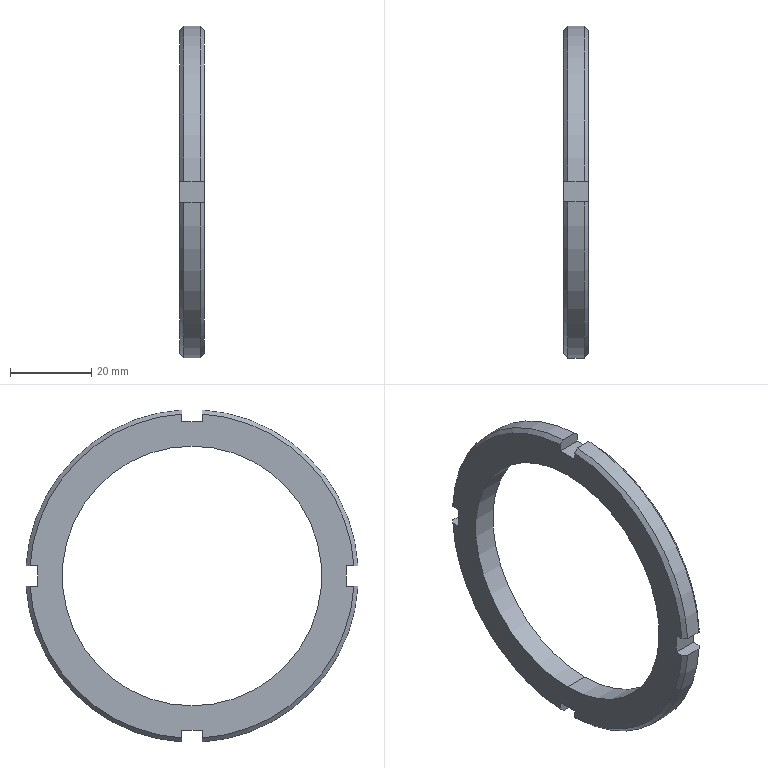Component | SolidWorks | 19LockNut-1 | 1 solid | 28 faces | box 6 x 81.85 x 81.85 mm | volume 11792 mm3 | plane 14 | cone 8 | cylinder 6 | commonest cylinder face diameters 82 x4 64 x2
build123d program:
from build123d import *

# Parameters (mm, degrees)
SKETCH9_R           = 41
BOSS_EXTRUDE3_DEPTH = 6
CHAMFER1_SIZE       = 1
SKETCH10_W          = 5
SKETCH10_H          = 19.557
CUT_EXTRUDE5_DEPTH  = 59.292
CIRPATTERN1_COUNT   = 4
M64_TAPPED_HOLE1_D  = 64


with BuildPart() as part:
    # Sketch9 → Boss-Extrude3 (new body)
    with BuildSketch(Plane(origin=(0, 0, 0), x_dir=(0, 0, -1), z_dir=(1, 0, 0))):
        Circle(SKETCH9_R)
    extrude(amount=BOSS_EXTRUDE3_DEPTH)

    # Chamfer1
    chamfer1_edges = [part.edges().sort_by_distance(p)[0] for p in [
        (0, 0, 41),
        (6, 0, 41),
    ]]
    chamfer(chamfer1_edges, length=CHAMFER1_SIZE)

    # Sketch10 → Cut-Extrude5 (cut, through all)
    with BuildSketch(Plane(origin=(6, 0, 0), x_dir=(0, 0, -1), z_dir=(1, 0, 0))):
        with Locations((0, 47.779)):
            Rectangle(SKETCH10_W, SKETCH10_H)
    cut_extrude5 = extrude(amount=-CUT_EXTRUDE5_DEPTH, mode=Mode.SUBTRACT)

    # CirPattern1: Cut-Extrude5 ×4 about axis
    cirpattern1_axis = Axis((0, 0, 0), (1, 0, 0))
    for i in range(1, CIRPATTERN1_COUNT):
        add(cut_extrude5.rotate(cirpattern1_axis, i * 360 / CIRPATTERN1_COUNT), mode=Mode.SUBTRACT)

    # M64 Tapped Hole1 (through all)
    with Locations(Plane(origin=(6, 0, 0), x_dir=(0, 0, -1), z_dir=(1, 0, 0))):
        with Locations((0, 0)):
            Hole(M64_TAPPED_HOLE1_D / 2)


solid = part.part

# Placed as in the assembly
solid = solid.moved(Location((-10.043, 1.776, 250), (0, 0, 0)))
STEP:
#1=CARTESIAN_POINT('',(-0.3954,0.06992,11.102));
#2=VERTEX_POINT('',#1);
#3=CARTESIAN_POINT('',(-0.3954,0.06992,8.583));
#4=VERTEX_POINT('',#3);
#5=CARTESIAN_POINT('',(-0.3954,0.06992,9.843));
#6=DIRECTION('',(1.,0.,0.));
#7=DIRECTION('',(0.,0.,-1.));
#8=AXIS2_PLACEMENT_3D('',#5,#6,#7);
#9=CIRCLE('',#8,1.26);
#10=EDGE_CURVE('',#2,#4,#9,.T.);
#11=ORIENTED_EDGE('',*,*,#10,.F.);
#12=CARTESIAN_POINT('',(-0.1592,0.06992,11.102));
#13=VERTEX_POINT('',#12);
#14=CARTESIAN_POINT('',(-0.1592,0.06992,11.102));
#15=DIRECTION('',(1.,0.,0.));
#16=VECTOR('',#15,39.37);
#17=LINE('',#14,#16);
#18=EDGE_CURVE('',#2,#13,#17,.T.);
#19=ORIENTED_EDGE('',*,*,#18,.T.);
#20=CARTESIAN_POINT('',(-0.1592,0.06992,8.583));
#21=VERTEX_POINT('',#20);
#22=CARTESIAN_POINT('',(-0.1592,0.06992,9.843));
#23=DIRECTION('',(1.,0.,0.));
#24=DIRECTION('',(0.,0.,-1.));
#25=AXIS2_PLACEMENT_3D('',#22,#23,#24);
#26=CIRCLE('',#25,1.26);
#27=EDGE_CURVE('',#13,#21,#26,.T.);
#28=ORIENTED_EDGE('',*,*,#27,.T.);
#29=CARTESIAN_POINT('',(-0.1592,0.06992,8.583));
#30=DIRECTION('',(1.,0.,0.));
#31=VECTOR('',#30,39.37);
#32=LINE('',#29,#31);
#33=EDGE_CURVE('',#4,#21,#32,.T.);
#34=ORIENTED_EDGE('',*,*,#33,.F.);
#35=EDGE_LOOP('',(#11,#19,#28,#34));
#36=FACE_OUTER_BOUND('',#35,.T.);
#37=CARTESIAN_POINT('',(-0.1592,0.06992,9.843));
#38=DIRECTION('',(1.,0.,0.));
#39=DIRECTION('',(0.,0.,-1.));
#40=AXIS2_PLACEMENT_3D('',#37,#38,#39);
#41=CYLINDRICAL_SURFACE('',#40,1.26);
#42=ADVANCED_FACE('',(#36),#41,.F.);
#43=CARTESIAN_POINT('',(-0.356,1.681,9.941));
#44=VERTEX_POINT('',#43);
#45=CARTESIAN_POINT('',(-0.356,0.1683,11.454));
#46=VERTEX_POINT('',#45);
#47=CARTESIAN_POINT('',(-0.356,0.06992,9.843));
#48=DIRECTION('',(1.,0.,0.));
#49=DIRECTION('',(0.,0.,-1.));
#50=AXIS2_PLACEMENT_3D('',#47,#48,#49);
#51=CIRCLE('',#50,1.614);
#52=EDGE_CURVE('',#44,#46,#51,.T.);
#53=ORIENTED_EDGE('',*,*,#52,.T.);
#54=CARTESIAN_POINT('',(-0.1985,0.1683,11.454));
#55=VERTEX_POINT('',#54);
#56=CARTESIAN_POINT('',(-0.1592,0.1683,11.454));
#57=DIRECTION('',(1.,0.,0.));
#58=VECTOR('',#57,39.37);
#59=LINE('',#56,#58);
#60=EDGE_CURVE('',#46,#55,#59,.T.);
#61=ORIENTED_EDGE('',*,*,#60,.T.);
#62=CARTESIAN_POINT('',(-0.1985,1.681,9.941));
#63=VERTEX_POINT('',#62);
#64=CARTESIAN_POINT('',(-0.1985,0.06992,9.843));
#65=DIRECTION('',(-1.,0.,0.));
#66=DIRECTION('',(0.,0.,-1.));
#67=AXIS2_PLACEMENT_3D('',#64,#65,#66);
#68=CIRCLE('',#67,1.614);
#69=EDGE_CURVE('',#55,#63,#68,.T.);
#70=ORIENTED_EDGE('',*,*,#69,.T.);
#71=CARTESIAN_POINT('',(-0.1592,1.681,9.941));
#72=DIRECTION('',(-1.,0.,0.));
#73=VECTOR('',#72,39.37);
#74=LINE('',#71,#73);
#75=EDGE_CURVE('',#63,#44,#74,.T.);
#76=ORIENTED_EDGE('',*,*,#75,.T.);
#77=EDGE_LOOP('',(#53,#61,#70,#76));
#78=FACE_OUTER_BOUND('',#77,.T.);
#79=CARTESIAN_POINT('',(-0.1592,0.06992,9.843));
#80=DIRECTION('',(-1.,0.,0.));
#81=DIRECTION('',(0.,0.,1.));
#82=AXIS2_PLACEMENT_3D('',#79,#80,#81);
#83=CYLINDRICAL_SURFACE('',#82,1.614);
#84=ADVANCED_FACE('',(#78),#83,.T.);
#85=CARTESIAN_POINT('',(-0.1985,-1.541,9.941));
#86=VERTEX_POINT('',#85);
#87=CARTESIAN_POINT('',(-0.1985,-0.0285,11.454));
#88=VERTEX_POINT('',#87);
#89=CARTESIAN_POINT('',(-0.1985,0.06992,9.843));
#90=DIRECTION('',(-1.,0.,0.));
#91=DIRECTION('',(0.,-0.,-1.));
#92=AXIS2_PLACEMENT_3D('',#89,#90,#91);
#93=CIRCLE('',#92,1.614);
#94=EDGE_CURVE('',#86,#88,#93,.T.);
#95=ORIENTED_EDGE('',*,*,#94,.T.);
#96=CARTESIAN_POINT('',(-0.356,-0.0285,11.454));
#97=VERTEX_POINT('',#96);
#98=CARTESIAN_POINT('',(-0.1592,-0.0285,11.454));
#99=DIRECTION('',(-1.,0.,0.));
#100=VECTOR('',#99,39.37);
#101=LINE('',#98,#100);
#102=EDGE_CURVE('',#88,#97,#101,.T.);
#103=ORIENTED_EDGE('',*,*,#102,.T.);
#104=CARTESIAN_POINT('',(-0.356,-1.541,9.941));
#105=VERTEX_POINT('',#104);
#106=CARTESIAN_POINT('',(-0.356,0.06992,9.843));
#107=DIRECTION('',(1.,0.,0.));
#108=DIRECTION('',(0.,0.,-1.));
#109=AXIS2_PLACEMENT_3D('',#106,#107,#108);
#110=CIRCLE('',#109,1.614);
#111=EDGE_CURVE('',#97,#105,#110,.T.);
#112=ORIENTED_EDGE('',*,*,#111,.T.);
#113=CARTESIAN_POINT('',(-0.1592,-1.541,9.941));
#114=DIRECTION('',(1.,0.,0.));
#115=VECTOR('',#114,39.37);
#116=LINE('',#113,#115);
#117=EDGE_CURVE('',#105,#86,#116,.T.);
#118=ORIENTED_EDGE('',*,*,#117,.T.);
#119=EDGE_LOOP('',(#95,#103,#112,#118));
#120=FACE_OUTER_BOUND('',#119,.T.);
#121=CARTESIAN_POINT('',(-0.1592,0.06992,9.843));
#122=DIRECTION('',(-1.,0.,0.));
#123=DIRECTION('',(0.,0.,1.));
#124=AXIS2_PLACEMENT_3D('',#121,#122,#123);
#125=CYLINDRICAL_SURFACE('',#124,1.614);
#126=ADVANCED_FACE('',(#120),#125,.T.);
#127=CARTESIAN_POINT('',(-0.1985,-0.0285,8.231));
#128=VERTEX_POINT('',#127);
#129=CARTESIAN_POINT('',(-0.1985,-1.541,9.744));
#130=VERTEX_POINT('',#129);
#131=CARTESIAN_POINT('',(-0.1985,0.06992,9.843));
#132=DIRECTION('',(-1.,0.,0.));
#133=DIRECTION('',(0.,0.,-1.));
#134=AXIS2_PLACEMENT_3D('',#131,#132,#133);
#135=CIRCLE('',#134,1.614);
#136=EDGE_CURVE('',#128,#130,#135,.T.);
#137=ORIENTED_EDGE('',*,*,#136,.T.);
#138=CARTESIAN_POINT('',(-0.356,-1.541,9.744));
#139=VERTEX_POINT('',#138);
#140=CARTESIAN_POINT('',(-0.1592,-1.541,9.744));
#141=DIRECTION('',(-1.,0.,0.));
#142=VECTOR('',#141,39.37);
#143=LINE('',#140,#142);
#144=EDGE_CURVE('',#130,#139,#143,.T.);
#145=ORIENTED_EDGE('',*,*,#144,.T.);
#146=CARTESIAN_POINT('',(-0.356,-0.0285,8.231));
#147=VERTEX_POINT('',#146);
#148=CARTESIAN_POINT('',(-0.356,0.06992,9.843));
#149=DIRECTION('',(1.,0.,0.));
#150=DIRECTION('',(0.,0.,-1.));
#151=AXIS2_PLACEMENT_3D('',#148,#149,#150);
#152=CIRCLE('',#151,1.614);
#153=EDGE_CURVE('',#139,#147,#152,.T.);
#154=ORIENTED_EDGE('',*,*,#153,.T.);
#155=CARTESIAN_POINT('',(-0.1592,-0.0285,8.231));
#156=DIRECTION('',(1.,0.,0.));
#157=VECTOR('',#156,39.37);
#158=LINE('',#155,#157);
#159=EDGE_CURVE('',#147,#128,#158,.T.);
#160=ORIENTED_EDGE('',*,*,#159,.T.);
#161=EDGE_LOOP('',(#137,#145,#154,#160));
#162=FACE_OUTER_BOUND('',#161,.T.);
#163=CARTESIAN_POINT('',(-0.1592,0.06992,9.843));
#164=DIRECTION('',(-1.,0.,0.));
#165=DIRECTION('',(0.,0.,1.));
#166=AXIS2_PLACEMENT_3D('',#163,#164,#165);
#167=CYLINDRICAL_SURFACE('',#166,1.614);
#168=ADVANCED_FACE('',(#162),#167,.T.);
#169=CARTESIAN_POINT('',(-0.3954,0.1683,11.414));
#170=VERTEX_POINT('',#169);
#171=CARTESIAN_POINT('',(-0.356,0.1683,11.454));
#172=CARTESIAN_POINT('',(-0.3662,0.1683,11.444));
#173=CARTESIAN_POINT('',(-0.3763,0.1683,11.433));
#174=CARTESIAN_POINT('',(-0.3865,0.1683,11.423));
#175=CARTESIAN_POINT('',(-0.3894,0.1683,11.42));
#176=CARTESIAN_POINT('',(-0.3924,0.1683,11.417));
#177=CARTESIAN_POINT('',(-0.3954,0.1683,11.414));
#178=B_SPLINE_CURVE_WITH_KNOTS('',3,(#171,#172,#173,#174,#175,#176,#177),.UNSPECIFIED.,.F.,.F.,(4,3,4),(0.005082,0.006177,0.006497),.UNSPECIFIED.);
#179=EDGE_CURVE('',#46,#170,#178,.T.);
#180=ORIENTED_EDGE('',*,*,#179,.F.);
#181=ORIENTED_EDGE('',*,*,#52,.F.);
#182=CARTESIAN_POINT('',(-0.3954,1.642,9.941));
#183=VERTEX_POINT('',#182);
#184=CARTESIAN_POINT('',(-0.3954,1.642,9.941));
#185=CARTESIAN_POINT('',(-0.3924,1.645,9.941));
#186=CARTESIAN_POINT('',(-0.3894,1.648,9.941));
#187=CARTESIAN_POINT('',(-0.3865,1.651,9.941));
#188=CARTESIAN_POINT('',(-0.3763,1.661,9.941));
#189=CARTESIAN_POINT('',(-0.3662,1.671,9.941));
#190=CARTESIAN_POINT('',(-0.356,1.681,9.941));
#191=B_SPLINE_CURVE_WITH_KNOTS('',3,(#184,#185,#186,#187,#188,#189,#190),.UNSPECIFIED.,.F.,.F.,(4,3,4),(0.005857,0.006177,0.007273),.UNSPECIFIED.);
#192=EDGE_CURVE('',#183,#44,#191,.T.);
#193=ORIENTED_EDGE('',*,*,#192,.F.);
#194=CARTESIAN_POINT('',(-0.3954,0.06992,9.843));
#195=DIRECTION('',(-1.,0.,0.));
#196=DIRECTION('',(0.,-0.,-1.));
#197=AXIS2_PLACEMENT_3D('',#194,#195,#196);
#198=CIRCLE('',#197,1.575);
#199=EDGE_CURVE('',#170,#183,#198,.T.);
#200=ORIENTED_EDGE('',*,*,#199,.F.);
#201=EDGE_LOOP('',(#180,#181,#193,#200));
#202=FACE_OUTER_BOUND('',#201,.T.);
#203=CARTESIAN_POINT('',(-0.356,0.06992,9.843));
#204=DIRECTION('',(1.,0.,0.));
#205=DIRECTION('',(0.,0.,-1.));
#206=AXIS2_PLACEMENT_3D('',#203,#204,#205);
#207=CONICAL_SURFACE('',#206,1.614,0.7854);
#208=ADVANCED_FACE('',(#202),#207,.T.);
#209=CARTESIAN_POINT('',(-0.3954,-0.0285,11.414));
#210=VERTEX_POINT('',#209);
#211=CARTESIAN_POINT('',(-0.3954,-0.0285,11.414));
#212=CARTESIAN_POINT('',(-0.3924,-0.0285,11.417));
#213=CARTESIAN_POINT('',(-0.3894,-0.0285,11.42));
#214=CARTESIAN_POINT('',(-0.3865,-0.0285,11.423));
#215=CARTESIAN_POINT('',(-0.3763,-0.0285,11.433));
#216=CARTESIAN_POINT('',(-0.3662,-0.0285,11.444));
#217=CARTESIAN_POINT('',(-0.356,-0.0285,11.454));
#218=B_SPLINE_CURVE_WITH_KNOTS('',3,(#211,#212,#213,#214,#215,#216,#217),.UNSPECIFIED.,.F.,.F.,(4,3,4),(0.005857,0.006177,0.007273),.UNSPECIFIED.);
#219=EDGE_CURVE('',#210,#97,#218,.T.);
#220=ORIENTED_EDGE('',*,*,#219,.F.);
#221=CARTESIAN_POINT('',(-0.3954,-1.502,9.941));
#222=VERTEX_POINT('',#221);
#223=CARTESIAN_POINT('',(-0.3954,0.06992,9.843));
#224=DIRECTION('',(-1.,0.,0.));
#225=DIRECTION('',(0.,0.,-1.));
#226=AXIS2_PLACEMENT_3D('',#223,#224,#225);
#227=CIRCLE('',#226,1.575);
#228=EDGE_CURVE('',#222,#210,#227,.T.);
#229=ORIENTED_EDGE('',*,*,#228,.F.);
#230=CARTESIAN_POINT('',(-0.356,-1.541,9.941));
#231=CARTESIAN_POINT('',(-0.3612,-1.536,9.941));
#232=CARTESIAN_POINT('',(-0.3665,-1.531,9.941));
#233=CARTESIAN_POINT('',(-0.3717,-1.526,9.941));
#234=CARTESIAN_POINT('',(-0.3796,-1.518,9.941));
#235=CARTESIAN_POINT('',(-0.3875,-1.51,9.941));
#236=CARTESIAN_POINT('',(-0.3954,-1.502,9.941));
#237=B_SPLINE_CURVE_WITH_KNOTS('',3,(#230,#231,#232,#233,#234,#235,#236),.UNSPECIFIED.,.F.,.F.,(4,3,4),(0.005613,0.006177,0.007028),.UNSPECIFIED.);
#238=EDGE_CURVE('',#105,#222,#237,.T.);
#239=ORIENTED_EDGE('',*,*,#238,.F.);
#240=ORIENTED_EDGE('',*,*,#111,.F.);
#241=EDGE_LOOP('',(#220,#229,#239,#240));
#242=FACE_OUTER_BOUND('',#241,.T.);
#243=CARTESIAN_POINT('',(-0.356,0.06992,9.843));
#244=DIRECTION('',(1.,0.,0.));
#245=DIRECTION('',(0.,0.,-1.));
#246=AXIS2_PLACEMENT_3D('',#243,#244,#245);
#247=CONICAL_SURFACE('',#246,1.614,0.7854);
#248=ADVANCED_FACE('',(#242),#247,.T.);
#249=CARTESIAN_POINT('',(-0.3954,-1.502,9.744));
#250=VERTEX_POINT('',#249);
#251=CARTESIAN_POINT('',(-0.3954,-1.502,9.744));
#252=CARTESIAN_POINT('',(-0.3875,-1.51,9.744));
#253=CARTESIAN_POINT('',(-0.3796,-1.518,9.744));
#254=CARTESIAN_POINT('',(-0.3717,-1.526,9.744));
#255=CARTESIAN_POINT('',(-0.3665,-1.531,9.744));
#256=CARTESIAN_POINT('',(-0.3612,-1.536,9.744));
#257=CARTESIAN_POINT('',(-0.356,-1.541,9.744));
#258=B_SPLINE_CURVE_WITH_KNOTS('',3,(#251,#252,#253,#254,#255,#256,#257),.UNSPECIFIED.,.F.,.F.,(4,3,4),(0.005326,0.006177,0.006742),.UNSPECIFIED.);
#259=EDGE_CURVE('',#250,#139,#258,.T.);
#260=ORIENTED_EDGE('',*,*,#259,.F.);
#261=CARTESIAN_POINT('',(-0.3954,-0.0285,8.271));
#262=VERTEX_POINT('',#261);
#263=CARTESIAN_POINT('',(-0.3954,0.06992,9.843));
#264=DIRECTION('',(-1.,0.,0.));
#265=DIRECTION('',(0.,0.,-1.));
#266=AXIS2_PLACEMENT_3D('',#263,#264,#265);
#267=CIRCLE('',#266,1.575);
#268=EDGE_CURVE('',#262,#250,#267,.T.);
#269=ORIENTED_EDGE('',*,*,#268,.F.);
#270=CARTESIAN_POINT('',(-0.356,-0.0285,8.231));
#271=CARTESIAN_POINT('',(-0.3612,-0.0285,8.237));
#272=CARTESIAN_POINT('',(-0.3665,-0.0285,8.242));
#273=CARTESIAN_POINT('',(-0.3717,-0.0285,8.247));
#274=CARTESIAN_POINT('',(-0.3796,-0.0285,8.255));
#275=CARTESIAN_POINT('',(-0.3875,-0.0285,8.263));
#276=CARTESIAN_POINT('',(-0.3954,-0.0285,8.271));
#277=B_SPLINE_CURVE_WITH_KNOTS('',3,(#270,#271,#272,#273,#274,#275,#276),.UNSPECIFIED.,.F.,.F.,(4,3,4),(0.005613,0.006177,0.007028),.UNSPECIFIED.);
#278=EDGE_CURVE('',#147,#262,#277,.T.);
#279=ORIENTED_EDGE('',*,*,#278,.F.);
#280=ORIENTED_EDGE('',*,*,#153,.F.);
#281=EDGE_LOOP('',(#260,#269,#279,#280));
#282=FACE_OUTER_BOUND('',#281,.T.);
#283=CARTESIAN_POINT('',(-0.356,0.06992,9.843));
#284=DIRECTION('',(1.,0.,0.));
#285=DIRECTION('',(0.,0.,-1.));
#286=AXIS2_PLACEMENT_3D('',#283,#284,#285);
#287=CONICAL_SURFACE('',#286,1.614,0.7854);
#288=ADVANCED_FACE('',(#282),#287,.T.);
#289=CARTESIAN_POINT('',(-0.1592,0.1683,11.414));
#290=VERTEX_POINT('',#289);
#291=CARTESIAN_POINT('',(-0.1592,0.1683,11.414));
#292=CARTESIAN_POINT('',(-0.1621,0.1683,11.417));
#293=CARTESIAN_POINT('',(-0.1651,0.1683,11.42));
#294=CARTESIAN_POINT('',(-0.1681,0.1683,11.423));
#295=CARTESIAN_POINT('',(-0.1782,0.1683,11.433));
#296=CARTESIAN_POINT('',(-0.1884,0.1683,11.444));
#297=CARTESIAN_POINT('',(-0.1985,0.1683,11.454));
#298=B_SPLINE_CURVE_WITH_KNOTS('',3,(#291,#292,#293,#294,#295,#296,#297),.UNSPECIFIED.,.F.,.F.,(4,3,4),(0.005857,0.006177,0.007273),.UNSPECIFIED.);
#299=EDGE_CURVE('',#290,#55,#298,.T.);
#300=ORIENTED_EDGE('',*,*,#299,.F.);
#301=CARTESIAN_POINT('',(-0.1592,1.642,9.941));
#302=VERTEX_POINT('',#301);
#303=CARTESIAN_POINT('',(-0.1592,0.06992,9.843));
#304=DIRECTION('',(1.,0.,0.));
#305=DIRECTION('',(0.,0.,-1.));
#306=AXIS2_PLACEMENT_3D('',#303,#304,#305);
#307=CIRCLE('',#306,1.575);
#308=EDGE_CURVE('',#302,#290,#307,.T.);
#309=ORIENTED_EDGE('',*,*,#308,.F.);
#310=CARTESIAN_POINT('',(-0.1985,1.681,9.941));
#311=CARTESIAN_POINT('',(-0.1884,1.671,9.941));
#312=CARTESIAN_POINT('',(-0.1782,1.661,9.941));
#313=CARTESIAN_POINT('',(-0.1681,1.651,9.941));
#314=CARTESIAN_POINT('',(-0.1651,1.648,9.941));
#315=CARTESIAN_POINT('',(-0.1621,1.645,9.941));
#316=CARTESIAN_POINT('',(-0.1592,1.642,9.941));
#317=B_SPLINE_CURVE_WITH_KNOTS('',3,(#310,#311,#312,#313,#314,#315,#316),.UNSPECIFIED.,.F.,.F.,(4,3,4),(0.005082,0.006177,0.006497),.UNSPECIFIED.);
#318=EDGE_CURVE('',#63,#302,#317,.T.);
#319=ORIENTED_EDGE('',*,*,#318,.F.);
#320=ORIENTED_EDGE('',*,*,#69,.F.);
#321=EDGE_LOOP('',(#300,#309,#319,#320));
#322=FACE_OUTER_BOUND('',#321,.T.);
#323=CARTESIAN_POINT('',(-0.1592,0.06992,9.843));
#324=DIRECTION('',(-1.,0.,0.));
#325=DIRECTION('',(0.,0.,1.));
#326=AXIS2_PLACEMENT_3D('',#323,#324,#325);
#327=CONICAL_SURFACE('',#326,1.575,0.7854);
#328=ADVANCED_FACE('',(#322),#327,.T.);
#329=CARTESIAN_POINT('',(-0.1592,-0.0285,11.414));
#330=VERTEX_POINT('',#329);
#331=CARTESIAN_POINT('',(-0.1985,-0.0285,11.454));
#332=CARTESIAN_POINT('',(-0.1884,-0.0285,11.444));
#333=CARTESIAN_POINT('',(-0.1782,-0.0285,11.433));
#334=CARTESIAN_POINT('',(-0.1681,-0.0285,11.423));
#335=CARTESIAN_POINT('',(-0.1651,-0.0285,11.42));
#336=CARTESIAN_POINT('',(-0.1621,-0.0285,11.417));
#337=CARTESIAN_POINT('',(-0.1592,-0.0285,11.414));
#338=B_SPLINE_CURVE_WITH_KNOTS('',3,(#331,#332,#333,#334,#335,#336,#337),.UNSPECIFIED.,.F.,.F.,(4,3,4),(0.005082,0.006177,0.006497),.UNSPECIFIED.);
#339=EDGE_CURVE('',#88,#330,#338,.T.);
#340=ORIENTED_EDGE('',*,*,#339,.F.);
#341=ORIENTED_EDGE('',*,*,#94,.F.);
#342=CARTESIAN_POINT('',(-0.1592,-1.502,9.941));
#343=VERTEX_POINT('',#342);
#344=CARTESIAN_POINT('',(-0.1592,-1.502,9.941));
#345=CARTESIAN_POINT('',(-0.1671,-1.51,9.941));
#346=CARTESIAN_POINT('',(-0.1749,-1.518,9.941));
#347=CARTESIAN_POINT('',(-0.1828,-1.526,9.941));
#348=CARTESIAN_POINT('',(-0.1881,-1.531,9.941));
#349=CARTESIAN_POINT('',(-0.1933,-1.536,9.941));
#350=CARTESIAN_POINT('',(-0.1985,-1.541,9.941));
#351=B_SPLINE_CURVE_WITH_KNOTS('',3,(#344,#345,#346,#347,#348,#349,#350),.UNSPECIFIED.,.F.,.F.,(4,3,4),(0.005326,0.006177,0.006742),.UNSPECIFIED.);
#352=EDGE_CURVE('',#343,#86,#351,.T.);
#353=ORIENTED_EDGE('',*,*,#352,.F.);
#354=CARTESIAN_POINT('',(-0.1592,0.06992,9.843));
#355=DIRECTION('',(1.,0.,0.));
#356=DIRECTION('',(0.,0.,-1.));
#357=AXIS2_PLACEMENT_3D('',#354,#355,#356);
#358=CIRCLE('',#357,1.575);
#359=EDGE_CURVE('',#330,#343,#358,.T.);
#360=ORIENTED_EDGE('',*,*,#359,.F.);
#361=EDGE_LOOP('',(#340,#341,#353,#360));
#362=FACE_OUTER_BOUND('',#361,.T.);
#363=CARTESIAN_POINT('',(-0.1592,0.06992,9.843));
#364=DIRECTION('',(-1.,0.,0.));
#365=DIRECTION('',(0.,0.,1.));
#366=AXIS2_PLACEMENT_3D('',#363,#364,#365);
#367=CONICAL_SURFACE('',#366,1.575,0.7854);
#368=ADVANCED_FACE('',(#362),#367,.T.);
#369=CARTESIAN_POINT('',(-0.1592,-1.502,9.744));
#370=VERTEX_POINT('',#369);
#371=CARTESIAN_POINT('',(-0.1985,-1.541,9.744));
#372=CARTESIAN_POINT('',(-0.1933,-1.536,9.744));
#373=CARTESIAN_POINT('',(-0.1881,-1.531,9.744));
#374=CARTESIAN_POINT('',(-0.1828,-1.526,9.744));
#375=CARTESIAN_POINT('',(-0.1749,-1.518,9.744));
#376=CARTESIAN_POINT('',(-0.1671,-1.51,9.744));
#377=CARTESIAN_POINT('',(-0.1592,-1.502,9.744));
#378=B_SPLINE_CURVE_WITH_KNOTS('',3,(#371,#372,#373,#374,#375,#376,#377),.UNSPECIFIED.,.F.,.F.,(4,3,4),(0.005613,0.006177,0.007028),.UNSPECIFIED.);
#379=EDGE_CURVE('',#130,#370,#378,.T.);
#380=ORIENTED_EDGE('',*,*,#379,.F.);
#381=ORIENTED_EDGE('',*,*,#136,.F.);
#382=CARTESIAN_POINT('',(-0.1592,-0.0285,8.271));
#383=VERTEX_POINT('',#382);
#384=CARTESIAN_POINT('',(-0.1592,-0.0285,8.271));
#385=CARTESIAN_POINT('',(-0.1671,-0.0285,8.263));
#386=CARTESIAN_POINT('',(-0.1749,-0.0285,8.255));
#387=CARTESIAN_POINT('',(-0.1828,-0.0285,8.247));
#388=CARTESIAN_POINT('',(-0.1881,-0.0285,8.242));
#389=CARTESIAN_POINT('',(-0.1933,-0.0285,8.237));
#390=CARTESIAN_POINT('',(-0.1985,-0.0285,8.231));
#391=B_SPLINE_CURVE_WITH_KNOTS('',3,(#384,#385,#386,#387,#388,#389,#390),.UNSPECIFIED.,.F.,.F.,(4,3,4),(0.005326,0.006177,0.006742),.UNSPECIFIED.);
#392=EDGE_CURVE('',#383,#128,#391,.T.);
#393=ORIENTED_EDGE('',*,*,#392,.F.);
#394=CARTESIAN_POINT('',(-0.1592,0.06992,9.843));
#395=DIRECTION('',(1.,0.,0.));
#396=DIRECTION('',(0.,0.,-1.));
#397=AXIS2_PLACEMENT_3D('',#394,#395,#396);
#398=CIRCLE('',#397,1.575);
#399=EDGE_CURVE('',#370,#383,#398,.T.);
#400=ORIENTED_EDGE('',*,*,#399,.F.);
#401=EDGE_LOOP('',(#380,#381,#393,#400));
#402=FACE_OUTER_BOUND('',#401,.T.);
#403=CARTESIAN_POINT('',(-0.1592,0.06992,9.843));
#404=DIRECTION('',(-1.,0.,0.));
#405=DIRECTION('',(0.,0.,1.));
#406=AXIS2_PLACEMENT_3D('',#403,#404,#405);
#407=CONICAL_SURFACE('',#406,1.575,0.7854);
#408=ADVANCED_FACE('',(#402),#407,.T.);
#409=CARTESIAN_POINT('',(-0.1985,1.681,9.744));
#410=VERTEX_POINT('',#409);
#411=CARTESIAN_POINT('',(-0.1985,0.1683,8.231));
#412=VERTEX_POINT('',#411);
#413=CARTESIAN_POINT('',(-0.1985,0.06992,9.843));
#414=DIRECTION('',(-1.,0.,0.));
#415=DIRECTION('',(0.,-0.,-1.));
#416=AXIS2_PLACEMENT_3D('',#413,#414,#415);
#417=CIRCLE('',#416,1.614);
#418=EDGE_CURVE('',#410,#412,#417,.T.);
#419=ORIENTED_EDGE('',*,*,#418,.T.);
#420=CARTESIAN_POINT('',(-0.356,0.1683,8.231));
#421=VERTEX_POINT('',#420);
#422=CARTESIAN_POINT('',(-0.1592,0.1683,8.231));
#423=DIRECTION('',(-1.,0.,0.));
#424=VECTOR('',#423,39.37);
#425=LINE('',#422,#424);
#426=EDGE_CURVE('',#412,#421,#425,.T.);
#427=ORIENTED_EDGE('',*,*,#426,.T.);
#428=CARTESIAN_POINT('',(-0.356,1.681,9.744));
#429=VERTEX_POINT('',#428);
#430=CARTESIAN_POINT('',(-0.356,0.06992,9.843));
#431=DIRECTION('',(1.,0.,0.));
#432=DIRECTION('',(0.,0.,-1.));
#433=AXIS2_PLACEMENT_3D('',#430,#431,#432);
#434=CIRCLE('',#433,1.614);
#435=EDGE_CURVE('',#421,#429,#434,.T.);
#436=ORIENTED_EDGE('',*,*,#435,.T.);
#437=CARTESIAN_POINT('',(-0.1592,1.681,9.744));
#438=DIRECTION('',(1.,0.,0.));
#439=VECTOR('',#438,39.37);
#440=LINE('',#437,#439);
#441=EDGE_CURVE('',#429,#410,#440,.T.);
#442=ORIENTED_EDGE('',*,*,#441,.T.);
#443=EDGE_LOOP('',(#419,#427,#436,#442));
#444=FACE_OUTER_BOUND('',#443,.T.);
#445=CARTESIAN_POINT('',(-0.1592,0.06992,9.843));
#446=DIRECTION('',(-1.,0.,0.));
#447=DIRECTION('',(0.,0.,1.));
#448=AXIS2_PLACEMENT_3D('',#445,#446,#447);
#449=CYLINDRICAL_SURFACE('',#448,1.614);
#450=ADVANCED_FACE('',(#444),#449,.T.);
#451=CARTESIAN_POINT('',(-0.1592,0.06992,9.843));
#452=DIRECTION('',(1.,0.,0.));
#453=DIRECTION('',(0.,0.,-1.));
#454=AXIS2_PLACEMENT_3D('',#451,#452,#453);
#455=CIRCLE('',#454,1.26);
#456=EDGE_CURVE('',#21,#13,#455,.T.);
#457=ORIENTED_EDGE('',*,*,#456,.F.);
#458=ORIENTED_EDGE('',*,*,#27,.F.);
#459=EDGE_LOOP('',(#457,#458));
#460=FACE_BOUND('',#459,.T.);
#461=CARTESIAN_POINT('',(-0.1592,0.1683,11.339));
#462=VERTEX_POINT('',#461);
#463=CARTESIAN_POINT('',(-0.1592,0.1683,12.109));
#464=DIRECTION('',(0.,-0.,1.));
#465=VECTOR('',#464,39.37);
#466=LINE('',#463,#465);
#467=EDGE_CURVE('',#462,#290,#466,.T.);
#468=ORIENTED_EDGE('',*,*,#467,.F.);
#469=CARTESIAN_POINT('',(-0.1592,-0.0285,11.339));
#470=VERTEX_POINT('',#469);
#471=CARTESIAN_POINT('',(-0.1592,-0.0285,11.339));
#472=DIRECTION('',(0.,1.,0.));
#473=VECTOR('',#472,39.37);
#474=LINE('',#471,#473);
#475=EDGE_CURVE('',#470,#462,#474,.T.);
#476=ORIENTED_EDGE('',*,*,#475,.F.);
#477=CARTESIAN_POINT('',(-0.1592,-0.0285,12.109));
#478=DIRECTION('',(0.,0.,-1.));
#479=VECTOR('',#478,39.37);
#480=LINE('',#477,#479);
#481=EDGE_CURVE('',#330,#470,#480,.T.);
#482=ORIENTED_EDGE('',*,*,#481,.F.);
#483=ORIENTED_EDGE('',*,*,#359,.T.);
#484=CARTESIAN_POINT('',(-0.1592,-1.426,9.941));
#485=VERTEX_POINT('',#484);
#486=CARTESIAN_POINT('',(-0.1592,-2.196,9.941));
#487=DIRECTION('',(0.,-1.,0.));
#488=VECTOR('',#487,39.37);
#489=LINE('',#486,#488);
#490=EDGE_CURVE('',#485,#343,#489,.T.);
#491=ORIENTED_EDGE('',*,*,#490,.F.);
#492=CARTESIAN_POINT('',(-0.1592,-1.426,9.744));
#493=VERTEX_POINT('',#492);
#494=CARTESIAN_POINT('',(-0.1592,-1.426,9.744));
#495=DIRECTION('',(0.,0.,1.));
#496=VECTOR('',#495,39.37);
#497=LINE('',#494,#496);
#498=EDGE_CURVE('',#493,#485,#497,.T.);
#499=ORIENTED_EDGE('',*,*,#498,.F.);
#500=CARTESIAN_POINT('',(-0.1592,-2.196,9.744));
#501=DIRECTION('',(0.,1.,0.));
#502=VECTOR('',#501,39.37);
#503=LINE('',#500,#502);
#504=EDGE_CURVE('',#370,#493,#503,.T.);
#505=ORIENTED_EDGE('',*,*,#504,.F.);
#506=ORIENTED_EDGE('',*,*,#399,.T.);
#507=CARTESIAN_POINT('',(-0.1592,-0.0285,8.346));
#508=VERTEX_POINT('',#507);
#509=CARTESIAN_POINT('',(-0.1592,-0.0285,7.576));
#510=DIRECTION('',(0.,0.,-1.));
#511=VECTOR('',#510,39.37);
#512=LINE('',#509,#511);
#513=EDGE_CURVE('',#508,#383,#512,.T.);
#514=ORIENTED_EDGE('',*,*,#513,.F.);
#515=CARTESIAN_POINT('',(-0.1592,0.1683,8.346));
#516=VERTEX_POINT('',#515);
#517=CARTESIAN_POINT('',(-0.1592,0.1683,8.346));
#518=DIRECTION('',(0.,-1.,-0.));
#519=VECTOR('',#518,39.37);
#520=LINE('',#517,#519);
#521=EDGE_CURVE('',#516,#508,#520,.T.);
#522=ORIENTED_EDGE('',*,*,#521,.F.);
#523=CARTESIAN_POINT('',(-0.1592,0.1683,8.271));
#524=VERTEX_POINT('',#523);
#525=CARTESIAN_POINT('',(-0.1592,0.1683,7.576));
#526=DIRECTION('',(0.,-0.,1.));
#527=VECTOR('',#526,39.37);
#528=LINE('',#525,#527);
#529=EDGE_CURVE('',#524,#516,#528,.T.);
#530=ORIENTED_EDGE('',*,*,#529,.F.);
#531=CARTESIAN_POINT('',(-0.1592,1.642,9.744));
#532=VERTEX_POINT('',#531);
#533=CARTESIAN_POINT('',(-0.1592,0.06992,9.843));
#534=DIRECTION('',(1.,0.,0.));
#535=DIRECTION('',(0.,0.,-1.));
#536=AXIS2_PLACEMENT_3D('',#533,#534,#535);
#537=CIRCLE('',#536,1.575);
#538=EDGE_CURVE('',#524,#532,#537,.T.);
#539=ORIENTED_EDGE('',*,*,#538,.T.);
#540=CARTESIAN_POINT('',(-0.1592,1.566,9.744));
#541=VERTEX_POINT('',#540);
#542=CARTESIAN_POINT('',(-0.1592,2.336,9.744));
#543=DIRECTION('',(0.,1.,0.));
#544=VECTOR('',#543,39.37);
#545=LINE('',#542,#544);
#546=EDGE_CURVE('',#541,#532,#545,.T.);
#547=ORIENTED_EDGE('',*,*,#546,.F.);
#548=CARTESIAN_POINT('',(-0.1592,1.566,9.941));
#549=VERTEX_POINT('',#548);
#550=CARTESIAN_POINT('',(-0.1592,1.566,9.941));
#551=DIRECTION('',(0.,0.,-1.));
#552=VECTOR('',#551,39.37);
#553=LINE('',#550,#552);
#554=EDGE_CURVE('',#549,#541,#553,.T.);
#555=ORIENTED_EDGE('',*,*,#554,.F.);
#556=CARTESIAN_POINT('',(-0.1592,2.336,9.941));
#557=DIRECTION('',(0.,-1.,0.));
#558=VECTOR('',#557,39.37);
#559=LINE('',#556,#558);
#560=EDGE_CURVE('',#302,#549,#559,.T.);
#561=ORIENTED_EDGE('',*,*,#560,.F.);
#562=ORIENTED_EDGE('',*,*,#308,.T.);
#563=EDGE_LOOP('',(#468,#476,#482,#483,#491,#499,#505,#506,#514,#522,#530,#539,#547,#555,#561,#562));
#564=FACE_OUTER_BOUND('',#563,.T.);
#565=CARTESIAN_POINT('',(-0.1592,0.06992,9.843));
#566=DIRECTION('',(1.,0.,0.));
#567=DIRECTION('',(0.,0.,-1.));
#568=AXIS2_PLACEMENT_3D('',#565,#566,#567);
#569=PLANE('',#568);
#570=ADVANCED_FACE('',(#460,#564),#569,.T.);
#571=CARTESIAN_POINT('',(-0.3954,0.06992,9.843));
#572=DIRECTION('',(1.,0.,0.));
#573=DIRECTION('',(0.,0.,-1.));
#574=AXIS2_PLACEMENT_3D('',#571,#572,#573);
#575=CIRCLE('',#574,1.26);
#576=EDGE_CURVE('',#4,#2,#575,.T.);
#577=ORIENTED_EDGE('',*,*,#576,.T.);
#578=ORIENTED_EDGE('',*,*,#10,.T.);
#579=EDGE_LOOP('',(#577,#578));
#580=FACE_BOUND('',#579,.T.);
#581=CARTESIAN_POINT('',(-0.3954,-0.0285,11.339));
#582=VERTEX_POINT('',#581);
#583=CARTESIAN_POINT('',(-0.3954,0.1683,11.339));
#584=VERTEX_POINT('',#583);
#585=CARTESIAN_POINT('',(-0.3954,-0.0285,11.339));
#586=DIRECTION('',(0.,1.,0.));
#587=VECTOR('',#586,39.37);
#588=LINE('',#585,#587);
#589=EDGE_CURVE('',#582,#584,#588,.T.);
#590=ORIENTED_EDGE('',*,*,#589,.T.);
#591=CARTESIAN_POINT('',(-0.3954,0.1683,12.109));
#592=DIRECTION('',(0.,-0.,1.));
#593=VECTOR('',#592,39.37);
#594=LINE('',#591,#593);
#595=EDGE_CURVE('',#584,#170,#594,.T.);
#596=ORIENTED_EDGE('',*,*,#595,.T.);
#597=ORIENTED_EDGE('',*,*,#199,.T.);
#598=CARTESIAN_POINT('',(-0.3954,1.566,9.941));
#599=VERTEX_POINT('',#598);
#600=CARTESIAN_POINT('',(-0.3954,2.336,9.941));
#601=DIRECTION('',(0.,-1.,0.));
#602=VECTOR('',#601,39.37);
#603=LINE('',#600,#602);
#604=EDGE_CURVE('',#183,#599,#603,.T.);
#605=ORIENTED_EDGE('',*,*,#604,.T.);
#606=CARTESIAN_POINT('',(-0.3954,1.566,9.744));
#607=VERTEX_POINT('',#606);
#608=CARTESIAN_POINT('',(-0.3954,1.566,9.941));
#609=DIRECTION('',(0.,0.,-1.));
#610=VECTOR('',#609,39.37);
#611=LINE('',#608,#610);
#612=EDGE_CURVE('',#599,#607,#611,.T.);
#613=ORIENTED_EDGE('',*,*,#612,.T.);
#614=CARTESIAN_POINT('',(-0.3954,1.642,9.744));
#615=VERTEX_POINT('',#614);
#616=CARTESIAN_POINT('',(-0.3954,2.336,9.744));
#617=DIRECTION('',(0.,1.,0.));
#618=VECTOR('',#617,39.37);
#619=LINE('',#616,#618);
#620=EDGE_CURVE('',#607,#615,#619,.T.);
#621=ORIENTED_EDGE('',*,*,#620,.T.);
#622=CARTESIAN_POINT('',(-0.3954,0.1683,8.271));
#623=VERTEX_POINT('',#622);
#624=CARTESIAN_POINT('',(-0.3954,0.06992,9.843));
#625=DIRECTION('',(-1.,0.,0.));
#626=DIRECTION('',(0.,-0.,-1.));
#627=AXIS2_PLACEMENT_3D('',#624,#625,#626);
#628=CIRCLE('',#627,1.575);
#629=EDGE_CURVE('',#615,#623,#628,.T.);
#630=ORIENTED_EDGE('',*,*,#629,.T.);
#631=CARTESIAN_POINT('',(-0.3954,0.1683,8.346));
#632=VERTEX_POINT('',#631);
#633=CARTESIAN_POINT('',(-0.3954,0.1683,7.576));
#634=DIRECTION('',(0.,-0.,1.));
#635=VECTOR('',#634,39.37);
#636=LINE('',#633,#635);
#637=EDGE_CURVE('',#623,#632,#636,.T.);
#638=ORIENTED_EDGE('',*,*,#637,.T.);
#639=CARTESIAN_POINT('',(-0.3954,-0.0285,8.346));
#640=VERTEX_POINT('',#639);
#641=CARTESIAN_POINT('',(-0.3954,0.1683,8.346));
#642=DIRECTION('',(0.,-1.,-0.));
#643=VECTOR('',#642,39.37);
#644=LINE('',#641,#643);
#645=EDGE_CURVE('',#632,#640,#644,.T.);
#646=ORIENTED_EDGE('',*,*,#645,.T.);
#647=CARTESIAN_POINT('',(-0.3954,-0.0285,7.576));
#648=DIRECTION('',(0.,0.,-1.));
#649=VECTOR('',#648,39.37);
#650=LINE('',#647,#649);
#651=EDGE_CURVE('',#640,#262,#650,.T.);
#652=ORIENTED_EDGE('',*,*,#651,.T.);
#653=ORIENTED_EDGE('',*,*,#268,.T.);
#654=CARTESIAN_POINT('',(-0.3954,-1.426,9.744));
#655=VERTEX_POINT('',#654);
#656=CARTESIAN_POINT('',(-0.3954,-2.196,9.744));
#657=DIRECTION('',(0.,1.,0.));
#658=VECTOR('',#657,39.37);
#659=LINE('',#656,#658);
#660=EDGE_CURVE('',#250,#655,#659,.T.);
#661=ORIENTED_EDGE('',*,*,#660,.T.);
#662=CARTESIAN_POINT('',(-0.3954,-1.426,9.941));
#663=VERTEX_POINT('',#662);
#664=CARTESIAN_POINT('',(-0.3954,-1.426,9.744));
#665=DIRECTION('',(0.,0.,1.));
#666=VECTOR('',#665,39.37);
#667=LINE('',#664,#666);
#668=EDGE_CURVE('',#655,#663,#667,.T.);
#669=ORIENTED_EDGE('',*,*,#668,.T.);
#670=CARTESIAN_POINT('',(-0.3954,-2.196,9.941));
#671=DIRECTION('',(0.,-1.,0.));
#672=VECTOR('',#671,39.37);
#673=LINE('',#670,#672);
#674=EDGE_CURVE('',#663,#222,#673,.T.);
#675=ORIENTED_EDGE('',*,*,#674,.T.);
#676=ORIENTED_EDGE('',*,*,#228,.T.);
#677=CARTESIAN_POINT('',(-0.3954,-0.0285,12.109));
#678=DIRECTION('',(0.,0.,-1.));
#679=VECTOR('',#678,39.37);
#680=LINE('',#677,#679);
#681=EDGE_CURVE('',#210,#582,#680,.T.);
#682=ORIENTED_EDGE('',*,*,#681,.T.);
#683=EDGE_LOOP('',(#590,#596,#597,#605,#613,#621,#630,#638,#646,#652,#653,#661,#669,#675,#676,#682));
#684=FACE_OUTER_BOUND('',#683,.T.);
#685=CARTESIAN_POINT('',(-0.3954,0.06992,9.843));
#686=DIRECTION('',(1.,0.,0.));
#687=DIRECTION('',(0.,0.,-1.));
#688=AXIS2_PLACEMENT_3D('',#685,#686,#687);
#689=PLANE('',#688);
#690=ADVANCED_FACE('',(#580,#684),#689,.F.);
#691=CARTESIAN_POINT('',(-0.3954,0.1683,8.271));
#692=CARTESIAN_POINT('',(-0.3875,0.1683,8.263));
#693=CARTESIAN_POINT('',(-0.3796,0.1683,8.255));
#694=CARTESIAN_POINT('',(-0.3717,0.1683,8.247));
#695=CARTESIAN_POINT('',(-0.3665,0.1683,8.242));
#696=CARTESIAN_POINT('',(-0.3612,0.1683,8.237));
#697=CARTESIAN_POINT('',(-0.356,0.1683,8.231));
#698=B_SPLINE_CURVE_WITH_KNOTS('',3,(#691,#692,#693,#694,#695,#696,#697),.UNSPECIFIED.,.F.,.F.,(4,3,4),(0.005326,0.006177,0.006742),.UNSPECIFIED.);
#699=EDGE_CURVE('',#623,#421,#698,.T.);
#700=ORIENTED_EDGE('',*,*,#699,.F.);
#701=ORIENTED_EDGE('',*,*,#629,.F.);
#702=CARTESIAN_POINT('',(-0.356,1.681,9.744));
#703=CARTESIAN_POINT('',(-0.3662,1.671,9.744));
#704=CARTESIAN_POINT('',(-0.3763,1.661,9.744));
#705=CARTESIAN_POINT('',(-0.3865,1.651,9.744));
#706=CARTESIAN_POINT('',(-0.3894,1.648,9.744));
#707=CARTESIAN_POINT('',(-0.3924,1.645,9.744));
#708=CARTESIAN_POINT('',(-0.3954,1.642,9.744));
#709=B_SPLINE_CURVE_WITH_KNOTS('',3,(#702,#703,#704,#705,#706,#707,#708),.UNSPECIFIED.,.F.,.F.,(4,3,4),(0.005082,0.006177,0.006497),.UNSPECIFIED.);
#710=EDGE_CURVE('',#429,#615,#709,.T.);
#711=ORIENTED_EDGE('',*,*,#710,.F.);
#712=ORIENTED_EDGE('',*,*,#435,.F.);
#713=EDGE_LOOP('',(#700,#701,#711,#712));
#714=FACE_OUTER_BOUND('',#713,.T.);
#715=CARTESIAN_POINT('',(-0.356,0.06992,9.843));
#716=DIRECTION('',(1.,0.,0.));
#717=DIRECTION('',(0.,0.,-1.));
#718=AXIS2_PLACEMENT_3D('',#715,#716,#717);
#719=CONICAL_SURFACE('',#718,1.614,0.7854);
#720=ADVANCED_FACE('',(#714),#719,.T.);
#721=CARTESIAN_POINT('',(-0.1985,0.1683,8.231));
#722=CARTESIAN_POINT('',(-0.1933,0.1683,8.237));
#723=CARTESIAN_POINT('',(-0.1881,0.1683,8.242));
#724=CARTESIAN_POINT('',(-0.1828,0.1683,8.247));
#725=CARTESIAN_POINT('',(-0.1749,0.1683,8.255));
#726=CARTESIAN_POINT('',(-0.1671,0.1683,8.263));
#727=CARTESIAN_POINT('',(-0.1592,0.1683,8.271));
#728=B_SPLINE_CURVE_WITH_KNOTS('',3,(#721,#722,#723,#724,#725,#726,#727),.UNSPECIFIED.,.F.,.F.,(4,3,4),(0.005613,0.006177,0.007028),.UNSPECIFIED.);
#729=EDGE_CURVE('',#412,#524,#728,.T.);
#730=ORIENTED_EDGE('',*,*,#729,.F.);
#731=ORIENTED_EDGE('',*,*,#418,.F.);
#732=CARTESIAN_POINT('',(-0.1592,1.642,9.744));
#733=CARTESIAN_POINT('',(-0.1621,1.645,9.744));
#734=CARTESIAN_POINT('',(-0.1651,1.648,9.744));
#735=CARTESIAN_POINT('',(-0.1681,1.651,9.744));
#736=CARTESIAN_POINT('',(-0.1782,1.661,9.744));
#737=CARTESIAN_POINT('',(-0.1884,1.671,9.744));
#738=CARTESIAN_POINT('',(-0.1985,1.681,9.744));
#739=B_SPLINE_CURVE_WITH_KNOTS('',3,(#732,#733,#734,#735,#736,#737,#738),.UNSPECIFIED.,.F.,.F.,(4,3,4),(0.005857,0.006177,0.007273),.UNSPECIFIED.);
#740=EDGE_CURVE('',#532,#410,#739,.T.);
#741=ORIENTED_EDGE('',*,*,#740,.F.);
#742=ORIENTED_EDGE('',*,*,#538,.F.);
#743=EDGE_LOOP('',(#730,#731,#741,#742));
#744=FACE_OUTER_BOUND('',#743,.T.);
#745=CARTESIAN_POINT('',(-0.1592,0.06992,9.843));
#746=DIRECTION('',(-1.,0.,0.));
#747=DIRECTION('',(0.,0.,1.));
#748=AXIS2_PLACEMENT_3D('',#745,#746,#747);
#749=CONICAL_SURFACE('',#748,1.575,0.7854);
#750=ADVANCED_FACE('',(#744),#749,.T.);
#751=ORIENTED_EDGE('',*,*,#710,.T.);
#752=ORIENTED_EDGE('',*,*,#620,.F.);
#753=CARTESIAN_POINT('',(-0.3954,1.566,9.744));
#754=DIRECTION('',(1.,0.,0.));
#755=VECTOR('',#754,39.37);
#756=LINE('',#753,#755);
#757=EDGE_CURVE('',#607,#541,#756,.T.);
#758=ORIENTED_EDGE('',*,*,#757,.T.);
#759=ORIENTED_EDGE('',*,*,#546,.T.);
#760=ORIENTED_EDGE('',*,*,#740,.T.);
#761=ORIENTED_EDGE('',*,*,#441,.F.);
#762=EDGE_LOOP('',(#751,#752,#758,#759,#760,#761));
#763=FACE_OUTER_BOUND('',#762,.T.);
#764=CARTESIAN_POINT('',(-0.3954,2.336,9.744));
#765=DIRECTION('',(0.,0.,-1.));
#766=DIRECTION('',(-1.,0.,0.));
#767=AXIS2_PLACEMENT_3D('',#764,#765,#766);
#768=PLANE('',#767);
#769=ADVANCED_FACE('',(#763),#768,.F.);
#770=ORIENTED_EDGE('',*,*,#554,.T.);
#771=ORIENTED_EDGE('',*,*,#757,.F.);
#772=ORIENTED_EDGE('',*,*,#612,.F.);
#773=CARTESIAN_POINT('',(-0.3954,1.566,9.941));
#774=DIRECTION('',(1.,0.,0.));
#775=VECTOR('',#774,39.37);
#776=LINE('',#773,#775);
#777=EDGE_CURVE('',#599,#549,#776,.T.);
#778=ORIENTED_EDGE('',*,*,#777,.T.);
#779=EDGE_LOOP('',(#770,#771,#772,#778));
#780=FACE_OUTER_BOUND('',#779,.T.);
#781=CARTESIAN_POINT('',(-0.3954,1.566,9.941));
#782=DIRECTION('',(0.,-1.,0.));
#783=DIRECTION('',(0.,0.,-1.));
#784=AXIS2_PLACEMENT_3D('',#781,#782,#783);
#785=PLANE('',#784);
#786=ADVANCED_FACE('',(#780),#785,.F.);
#787=ORIENTED_EDGE('',*,*,#192,.T.);
#788=ORIENTED_EDGE('',*,*,#75,.F.);
#789=ORIENTED_EDGE('',*,*,#318,.T.);
#790=ORIENTED_EDGE('',*,*,#560,.T.);
#791=ORIENTED_EDGE('',*,*,#777,.F.);
#792=ORIENTED_EDGE('',*,*,#604,.F.);
#793=EDGE_LOOP('',(#787,#788,#789,#790,#791,#792));
#794=FACE_OUTER_BOUND('',#793,.T.);
#795=CARTESIAN_POINT('',(-0.3954,2.336,9.941));
#796=DIRECTION('',(0.,0.,1.));
#797=DIRECTION('',(1.,0.,0.));
#798=AXIS2_PLACEMENT_3D('',#795,#796,#797);
#799=PLANE('',#798);
#800=ADVANCED_FACE('',(#794),#799,.F.);
#801=ORIENTED_EDGE('',*,*,#278,.T.);
#802=ORIENTED_EDGE('',*,*,#651,.F.);
#803=CARTESIAN_POINT('',(-0.3954,-0.0285,8.346));
#804=DIRECTION('',(1.,0.,0.));
#805=VECTOR('',#804,39.37);
#806=LINE('',#803,#805);
#807=EDGE_CURVE('',#640,#508,#806,.T.);
#808=ORIENTED_EDGE('',*,*,#807,.T.);
#809=ORIENTED_EDGE('',*,*,#513,.T.);
#810=ORIENTED_EDGE('',*,*,#392,.T.);
#811=ORIENTED_EDGE('',*,*,#159,.F.);
#812=EDGE_LOOP('',(#801,#802,#808,#809,#810,#811));
#813=FACE_OUTER_BOUND('',#812,.T.);
#814=CARTESIAN_POINT('',(-0.3954,-0.0285,7.576));
#815=DIRECTION('',(0.,-1.,-0.));
#816=DIRECTION('',(0.,0.,-1.));
#817=AXIS2_PLACEMENT_3D('',#814,#815,#816);
#818=PLANE('',#817);
#819=ADVANCED_FACE('',(#813),#818,.F.);
#820=ORIENTED_EDGE('',*,*,#521,.T.);
#821=ORIENTED_EDGE('',*,*,#807,.F.);
#822=ORIENTED_EDGE('',*,*,#645,.F.);
#823=CARTESIAN_POINT('',(-0.3954,0.1683,8.346));
#824=DIRECTION('',(1.,0.,0.));
#825=VECTOR('',#824,39.37);
#826=LINE('',#823,#825);
#827=EDGE_CURVE('',#632,#516,#826,.T.);
#828=ORIENTED_EDGE('',*,*,#827,.T.);
#829=EDGE_LOOP('',(#820,#821,#822,#828));
#830=FACE_OUTER_BOUND('',#829,.T.);
#831=CARTESIAN_POINT('',(-0.3954,0.1683,8.346));
#832=DIRECTION('',(0.,-0.,1.));
#833=DIRECTION('',(0.,-1.,-0.));
#834=AXIS2_PLACEMENT_3D('',#831,#832,#833);
#835=PLANE('',#834);
#836=ADVANCED_FACE('',(#830),#835,.F.);
#837=ORIENTED_EDGE('',*,*,#699,.T.);
#838=ORIENTED_EDGE('',*,*,#426,.F.);
#839=ORIENTED_EDGE('',*,*,#729,.T.);
#840=ORIENTED_EDGE('',*,*,#529,.T.);
#841=ORIENTED_EDGE('',*,*,#827,.F.);
#842=ORIENTED_EDGE('',*,*,#637,.F.);
#843=EDGE_LOOP('',(#837,#838,#839,#840,#841,#842));
#844=FACE_OUTER_BOUND('',#843,.T.);
#845=CARTESIAN_POINT('',(-0.3954,0.1683,7.576));
#846=DIRECTION('',(0.,1.,0.));
#847=DIRECTION('',(0.,-0.,1.));
#848=AXIS2_PLACEMENT_3D('',#845,#846,#847);
#849=PLANE('',#848);
#850=ADVANCED_FACE('',(#844),#849,.F.);
#851=ORIENTED_EDGE('',*,*,#238,.T.);
#852=ORIENTED_EDGE('',*,*,#674,.F.);
#853=CARTESIAN_POINT('',(-0.3954,-1.426,9.941));
#854=DIRECTION('',(1.,0.,0.));
#855=VECTOR('',#854,39.37);
#856=LINE('',#853,#855);
#857=EDGE_CURVE('',#663,#485,#856,.T.);
#858=ORIENTED_EDGE('',*,*,#857,.T.);
#859=ORIENTED_EDGE('',*,*,#490,.T.);
#860=ORIENTED_EDGE('',*,*,#352,.T.);
#861=ORIENTED_EDGE('',*,*,#117,.F.);
#862=EDGE_LOOP('',(#851,#852,#858,#859,#860,#861));
#863=FACE_OUTER_BOUND('',#862,.T.);
#864=CARTESIAN_POINT('',(-0.3954,-2.196,9.941));
#865=DIRECTION('',(0.,0.,1.));
#866=DIRECTION('',(1.,0.,0.));
#867=AXIS2_PLACEMENT_3D('',#864,#865,#866);
#868=PLANE('',#867);
#869=ADVANCED_FACE('',(#863),#868,.F.);
#870=ORIENTED_EDGE('',*,*,#498,.T.);
#871=ORIENTED_EDGE('',*,*,#857,.F.);
#872=ORIENTED_EDGE('',*,*,#668,.F.);
#873=CARTESIAN_POINT('',(-0.3954,-1.426,9.744));
#874=DIRECTION('',(1.,0.,0.));
#875=VECTOR('',#874,39.37);
#876=LINE('',#873,#875);
#877=EDGE_CURVE('',#655,#493,#876,.T.);
#878=ORIENTED_EDGE('',*,*,#877,.T.);
#879=EDGE_LOOP('',(#870,#871,#872,#878));
#880=FACE_OUTER_BOUND('',#879,.T.);
#881=CARTESIAN_POINT('',(-0.3954,-1.426,9.744));
#882=DIRECTION('',(0.,1.,0.));
#883=DIRECTION('',(0.,0.,1.));
#884=AXIS2_PLACEMENT_3D('',#881,#882,#883);
#885=PLANE('',#884);
#886=ADVANCED_FACE('',(#880),#885,.F.);
#887=ORIENTED_EDGE('',*,*,#259,.T.);
#888=ORIENTED_EDGE('',*,*,#144,.F.);
#889=ORIENTED_EDGE('',*,*,#379,.T.);
#890=ORIENTED_EDGE('',*,*,#504,.T.);
#891=ORIENTED_EDGE('',*,*,#877,.F.);
#892=ORIENTED_EDGE('',*,*,#660,.F.);
#893=EDGE_LOOP('',(#887,#888,#889,#890,#891,#892));
#894=FACE_OUTER_BOUND('',#893,.T.);
#895=CARTESIAN_POINT('',(-0.3954,-2.196,9.744));
#896=DIRECTION('',(0.,0.,-1.));
#897=DIRECTION('',(-1.,0.,0.));
#898=AXIS2_PLACEMENT_3D('',#895,#896,#897);
#899=PLANE('',#898);
#900=ADVANCED_FACE('',(#894),#899,.F.);
#901=ORIENTED_EDGE('',*,*,#179,.T.);
#902=ORIENTED_EDGE('',*,*,#595,.F.);
#903=CARTESIAN_POINT('',(-0.3954,0.1683,11.339));
#904=DIRECTION('',(1.,0.,0.));
#905=VECTOR('',#904,39.37);
#906=LINE('',#903,#905);
#907=EDGE_CURVE('',#584,#462,#906,.T.);
#908=ORIENTED_EDGE('',*,*,#907,.T.);
#909=ORIENTED_EDGE('',*,*,#467,.T.);
#910=ORIENTED_EDGE('',*,*,#299,.T.);
#911=ORIENTED_EDGE('',*,*,#60,.F.);
#912=EDGE_LOOP('',(#901,#902,#908,#909,#910,#911));
#913=FACE_OUTER_BOUND('',#912,.T.);
#914=CARTESIAN_POINT('',(-0.3954,0.1683,12.109));
#915=DIRECTION('',(0.,1.,0.));
#916=DIRECTION('',(0.,-0.,1.));
#917=AXIS2_PLACEMENT_3D('',#914,#915,#916);
#918=PLANE('',#917);
#919=ADVANCED_FACE('',(#913),#918,.F.);
#920=ORIENTED_EDGE('',*,*,#475,.T.);
#921=ORIENTED_EDGE('',*,*,#907,.F.);
#922=ORIENTED_EDGE('',*,*,#589,.F.);
#923=CARTESIAN_POINT('',(-0.3954,-0.0285,11.339));
#924=DIRECTION('',(1.,0.,0.));
#925=VECTOR('',#924,39.37);
#926=LINE('',#923,#925);
#927=EDGE_CURVE('',#582,#470,#926,.T.);
#928=ORIENTED_EDGE('',*,*,#927,.T.);
#929=EDGE_LOOP('',(#920,#921,#922,#928));
#930=FACE_OUTER_BOUND('',#929,.T.);
#931=CARTESIAN_POINT('',(-0.3954,-0.0285,11.339));
#932=DIRECTION('',(0.,0.,-1.));
#933=DIRECTION('',(0.,1.,0.));
#934=AXIS2_PLACEMENT_3D('',#931,#932,#933);
#935=PLANE('',#934);
#936=ADVANCED_FACE('',(#930),#935,.F.);
#937=ORIENTED_EDGE('',*,*,#219,.T.);
#938=ORIENTED_EDGE('',*,*,#102,.F.);
#939=ORIENTED_EDGE('',*,*,#339,.T.);
#940=ORIENTED_EDGE('',*,*,#481,.T.);
#941=ORIENTED_EDGE('',*,*,#927,.F.);
#942=ORIENTED_EDGE('',*,*,#681,.F.);
#943=EDGE_LOOP('',(#937,#938,#939,#940,#941,#942));
#944=FACE_OUTER_BOUND('',#943,.T.);
#945=CARTESIAN_POINT('',(-0.3954,-0.0285,12.109));
#946=DIRECTION('',(0.,-1.,-0.));
#947=DIRECTION('',(0.,0.,-1.));
#948=AXIS2_PLACEMENT_3D('',#945,#946,#947);
#949=PLANE('',#948);
#950=ADVANCED_FACE('',(#944),#949,.F.);
#951=ORIENTED_EDGE('',*,*,#18,.F.);
#952=ORIENTED_EDGE('',*,*,#576,.F.);
#953=ORIENTED_EDGE('',*,*,#33,.T.);
#954=ORIENTED_EDGE('',*,*,#456,.T.);
#955=EDGE_LOOP('',(#951,#952,#953,#954));
#956=FACE_OUTER_BOUND('',#955,.T.);
#957=CARTESIAN_POINT('',(-0.1592,0.06992,9.843));
#958=DIRECTION('',(1.,0.,0.));
#959=DIRECTION('',(0.,0.,-1.));
#960=AXIS2_PLACEMENT_3D('',#957,#958,#959);
#961=CYLINDRICAL_SURFACE('',#960,1.26);
#962=ADVANCED_FACE('',(#956),#961,.F.);
#963=CLOSED_SHELL('',(#42,#84,#126,#168,#208,#248,#288,#328,#368,#408,#450,#570,#690,#720,#750,#769,#786,#800,#819,#836,#850,#869,#886,#900,#919,#936,#950,#962));
#964=MANIFOLD_SOLID_BREP('',#963);
#965=CARTESIAN_POINT('',(0.,0.,0.));
#966=DIRECTION('',(0.,0.,1.));
#967=DIRECTION('',(1.,0.,0.));
#968=AXIS2_PLACEMENT_3D('',#965,#966,#967);
#969=(LENGTH_UNIT()NAMED_UNIT(*)SI_UNIT($,.METRE.));
#970=LENGTH_MEASURE_WITH_UNIT(LENGTH_MEASURE(0.0254),#969);
#971=DIMENSIONAL_EXPONENTS(1.,0.,0.,0.,0.,0.,0.);
#972=(CONVERSION_BASED_UNIT('',#970)LENGTH_UNIT()NAMED_UNIT(#971));
#973=UNCERTAINTY_MEASURE_WITH_UNIT(LENGTH_MEASURE(0.00001),#972,'','');
#974=(NAMED_UNIT(*)PLANE_ANGLE_UNIT()SI_UNIT($,.RADIAN.));
#975=(NAMED_UNIT(*)SI_UNIT($,.STERADIAN.)SOLID_ANGLE_UNIT());
#976=(GEOMETRIC_REPRESENTATION_CONTEXT(3)GLOBAL_UNCERTAINTY_ASSIGNED_CONTEXT((#973))GLOBAL_UNIT_ASSIGNED_CONTEXT((#972,#974,#975))REPRESENTATION_CONTEXT('',''));
#977=ADVANCED_BREP_SHAPE_REPRESENTATION('',(#964,#968),#976);
#978=COLOUR_RGB('',0.7922,0.8196,0.9333);
#979=FILL_AREA_STYLE_COLOUR('',#978);
#980=FILL_AREA_STYLE('',(#979));
#981=SURFACE_STYLE_FILL_AREA(#980);
#982=SURFACE_SIDE_STYLE('',(#981));
#983=SURFACE_STYLE_USAGE(.BOTH.,#982);
#984=PRESENTATION_STYLE_ASSIGNMENT((#983));
#985=STYLED_ITEM('',(#984),#964);
#986=PRESENTATION_LAYER_ASSIGNMENT('','',(#985));
#987=(LENGTH_UNIT()NAMED_UNIT(*)SI_UNIT($,.METRE.));
#988=LENGTH_MEASURE_WITH_UNIT(LENGTH_MEASURE(0.0254),#987);
#989=DIMENSIONAL_EXPONENTS(1.,0.,0.,0.,0.,0.,0.);
#990=(CONVERSION_BASED_UNIT('',#988)LENGTH_UNIT()NAMED_UNIT(#989));
#991=UNCERTAINTY_MEASURE_WITH_UNIT(LENGTH_MEASURE(0.00001),#990,'','');
#992=(NAMED_UNIT(*)PLANE_ANGLE_UNIT()SI_UNIT($,.RADIAN.));
#993=(NAMED_UNIT(*)SI_UNIT($,.STERADIAN.)SOLID_ANGLE_UNIT());
#994=(GEOMETRIC_REPRESENTATION_CONTEXT(3)GLOBAL_UNCERTAINTY_ASSIGNED_CONTEXT((#991))GLOBAL_UNIT_ASSIGNED_CONTEXT((#990,#992,#993))REPRESENTATION_CONTEXT('',''));
#995=MECHANICAL_DESIGN_GEOMETRIC_PRESENTATION_REPRESENTATION('',(#985),#994);